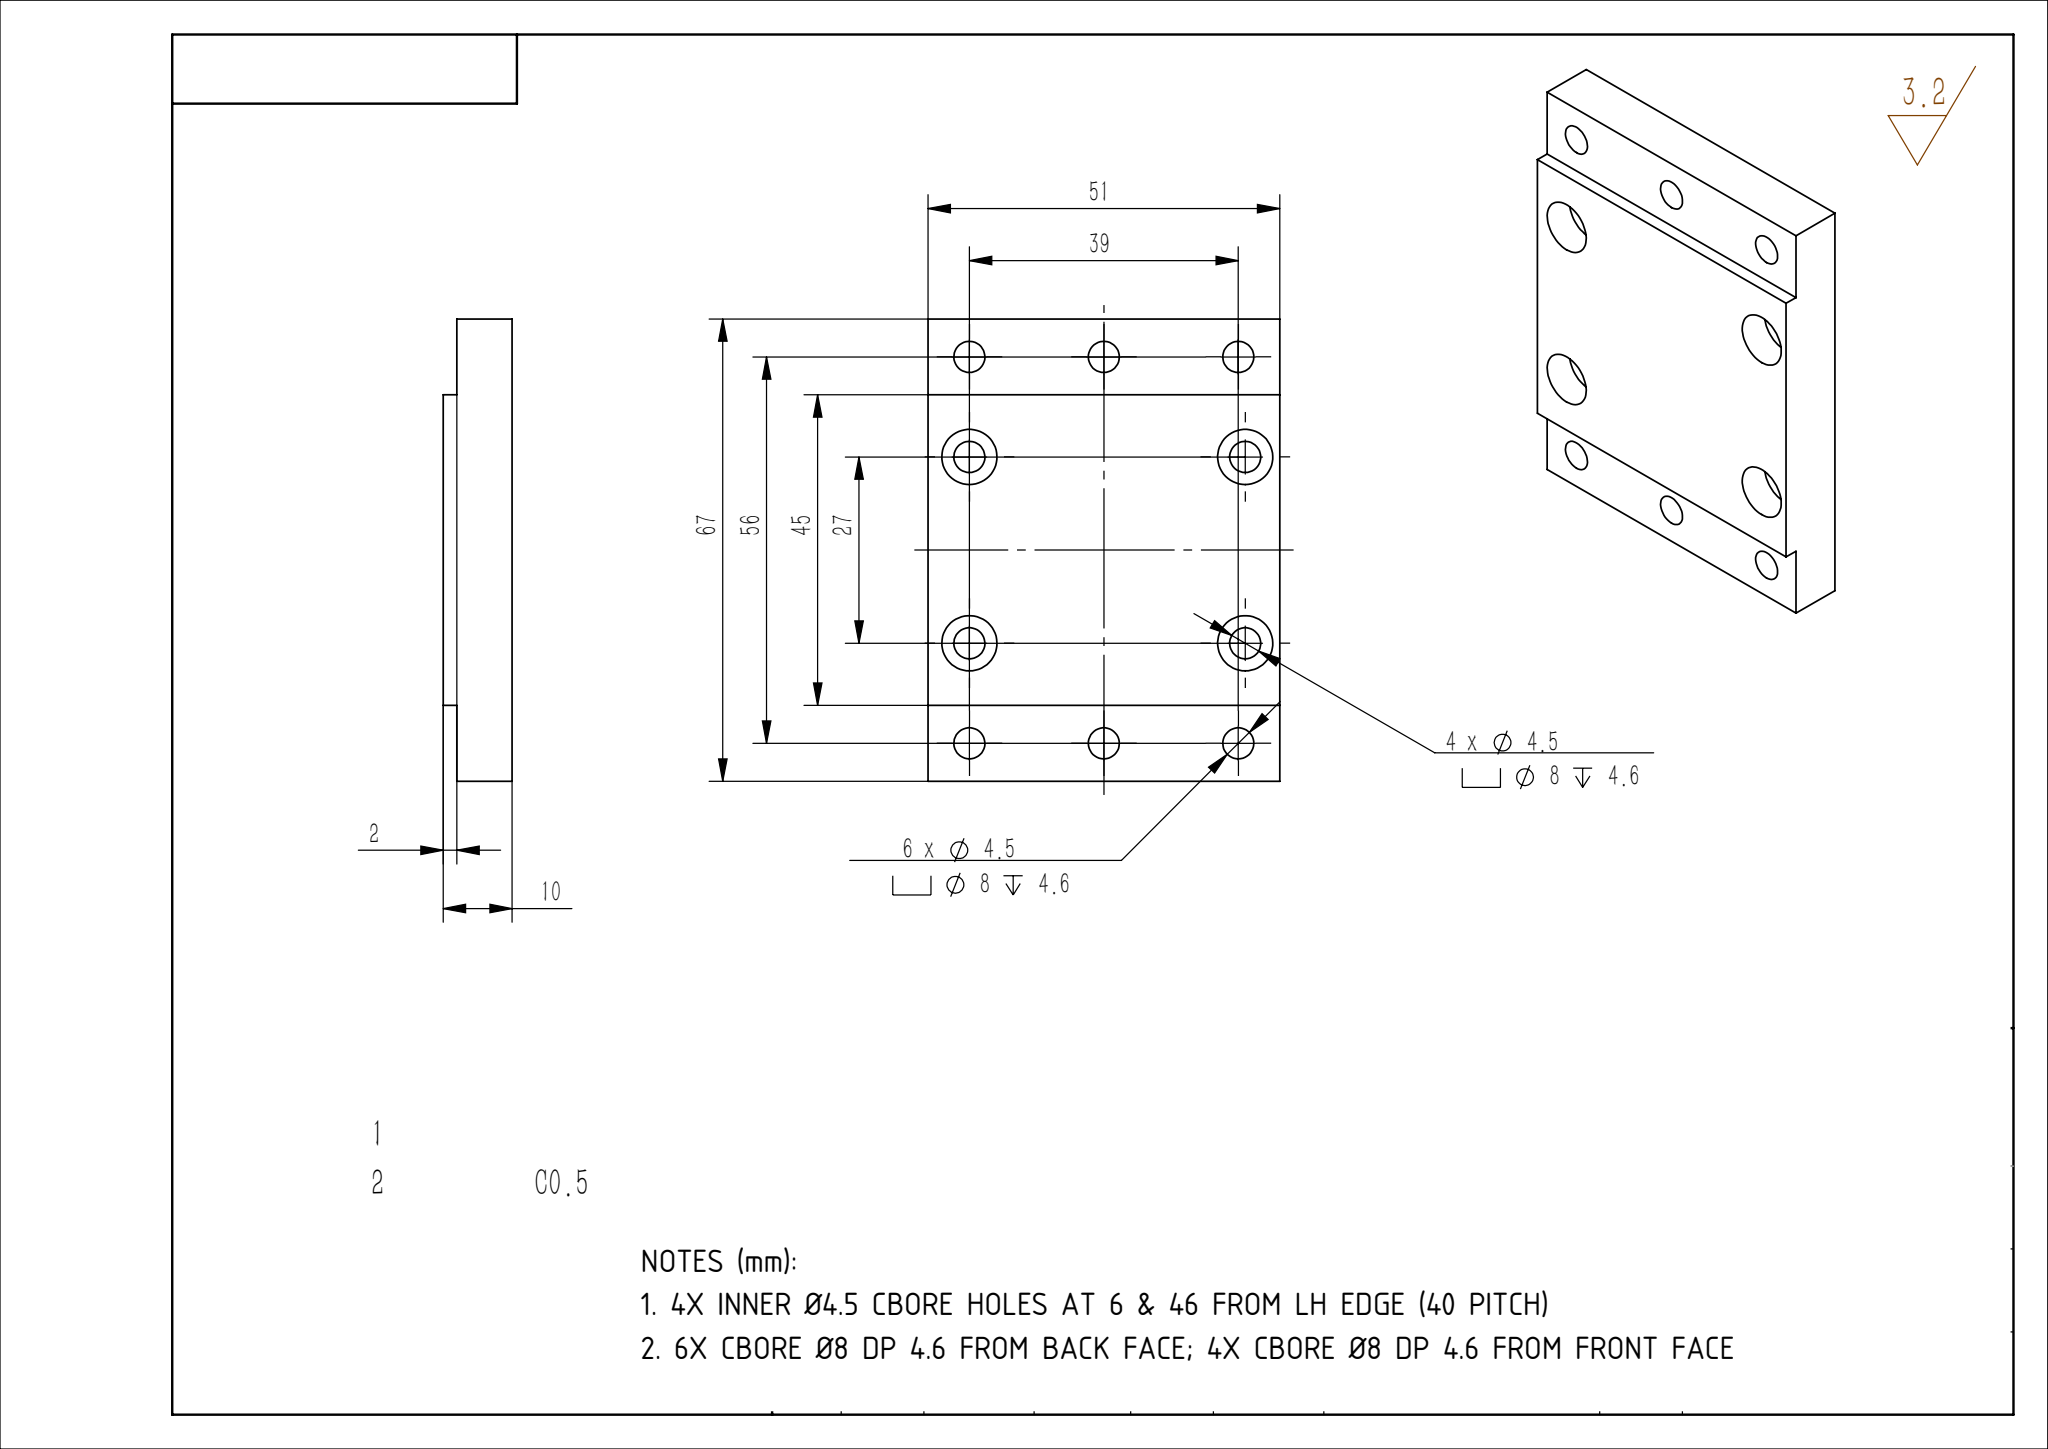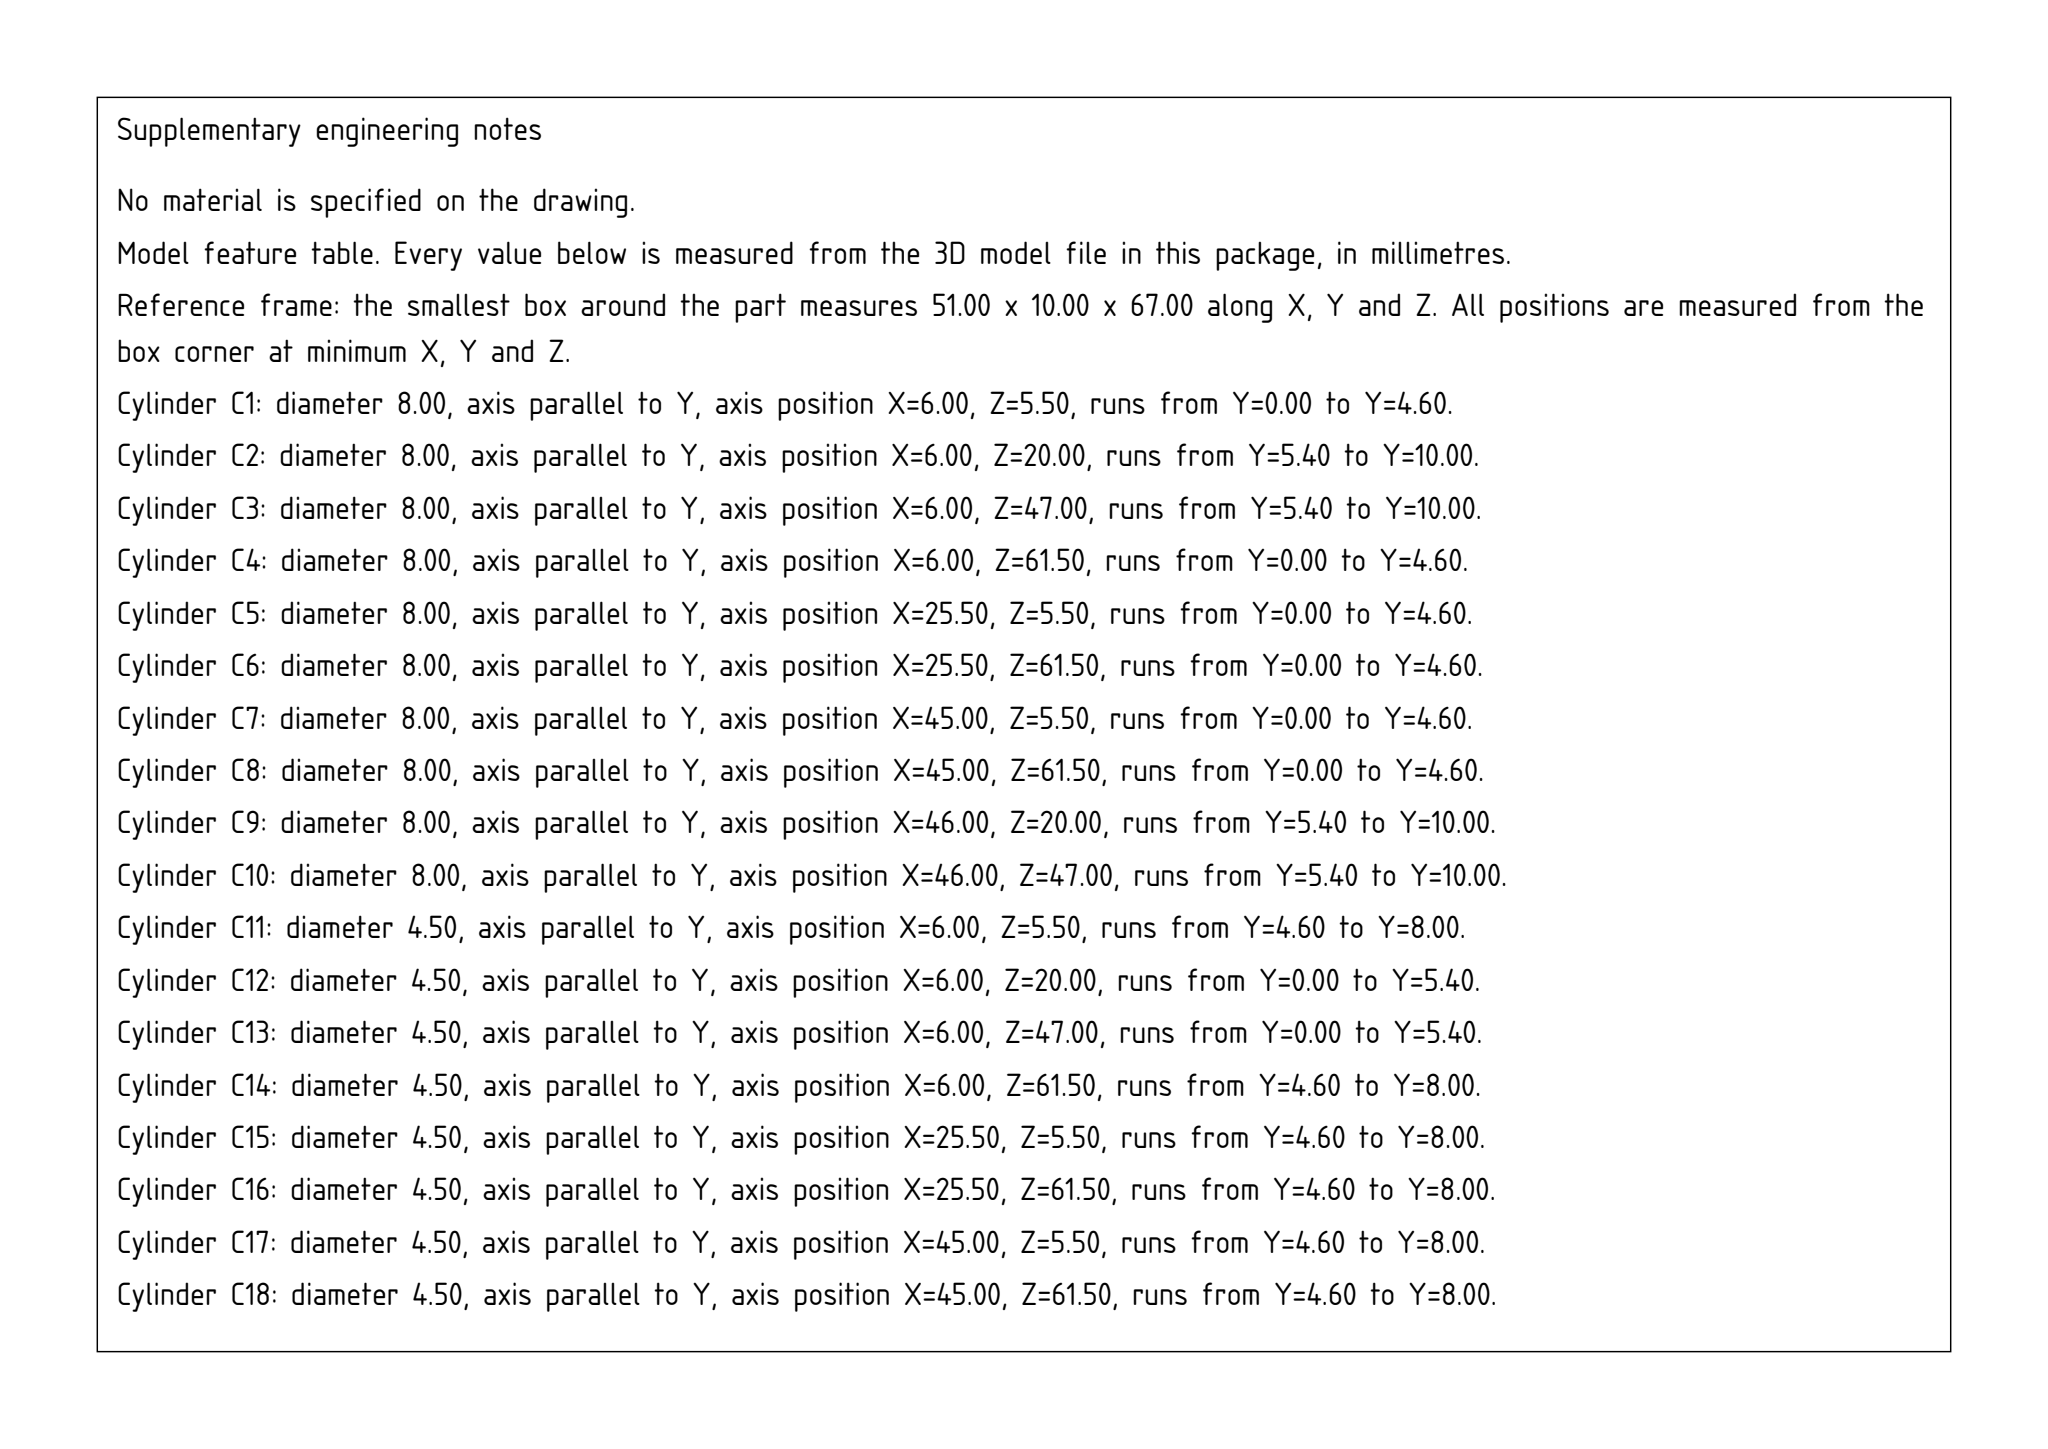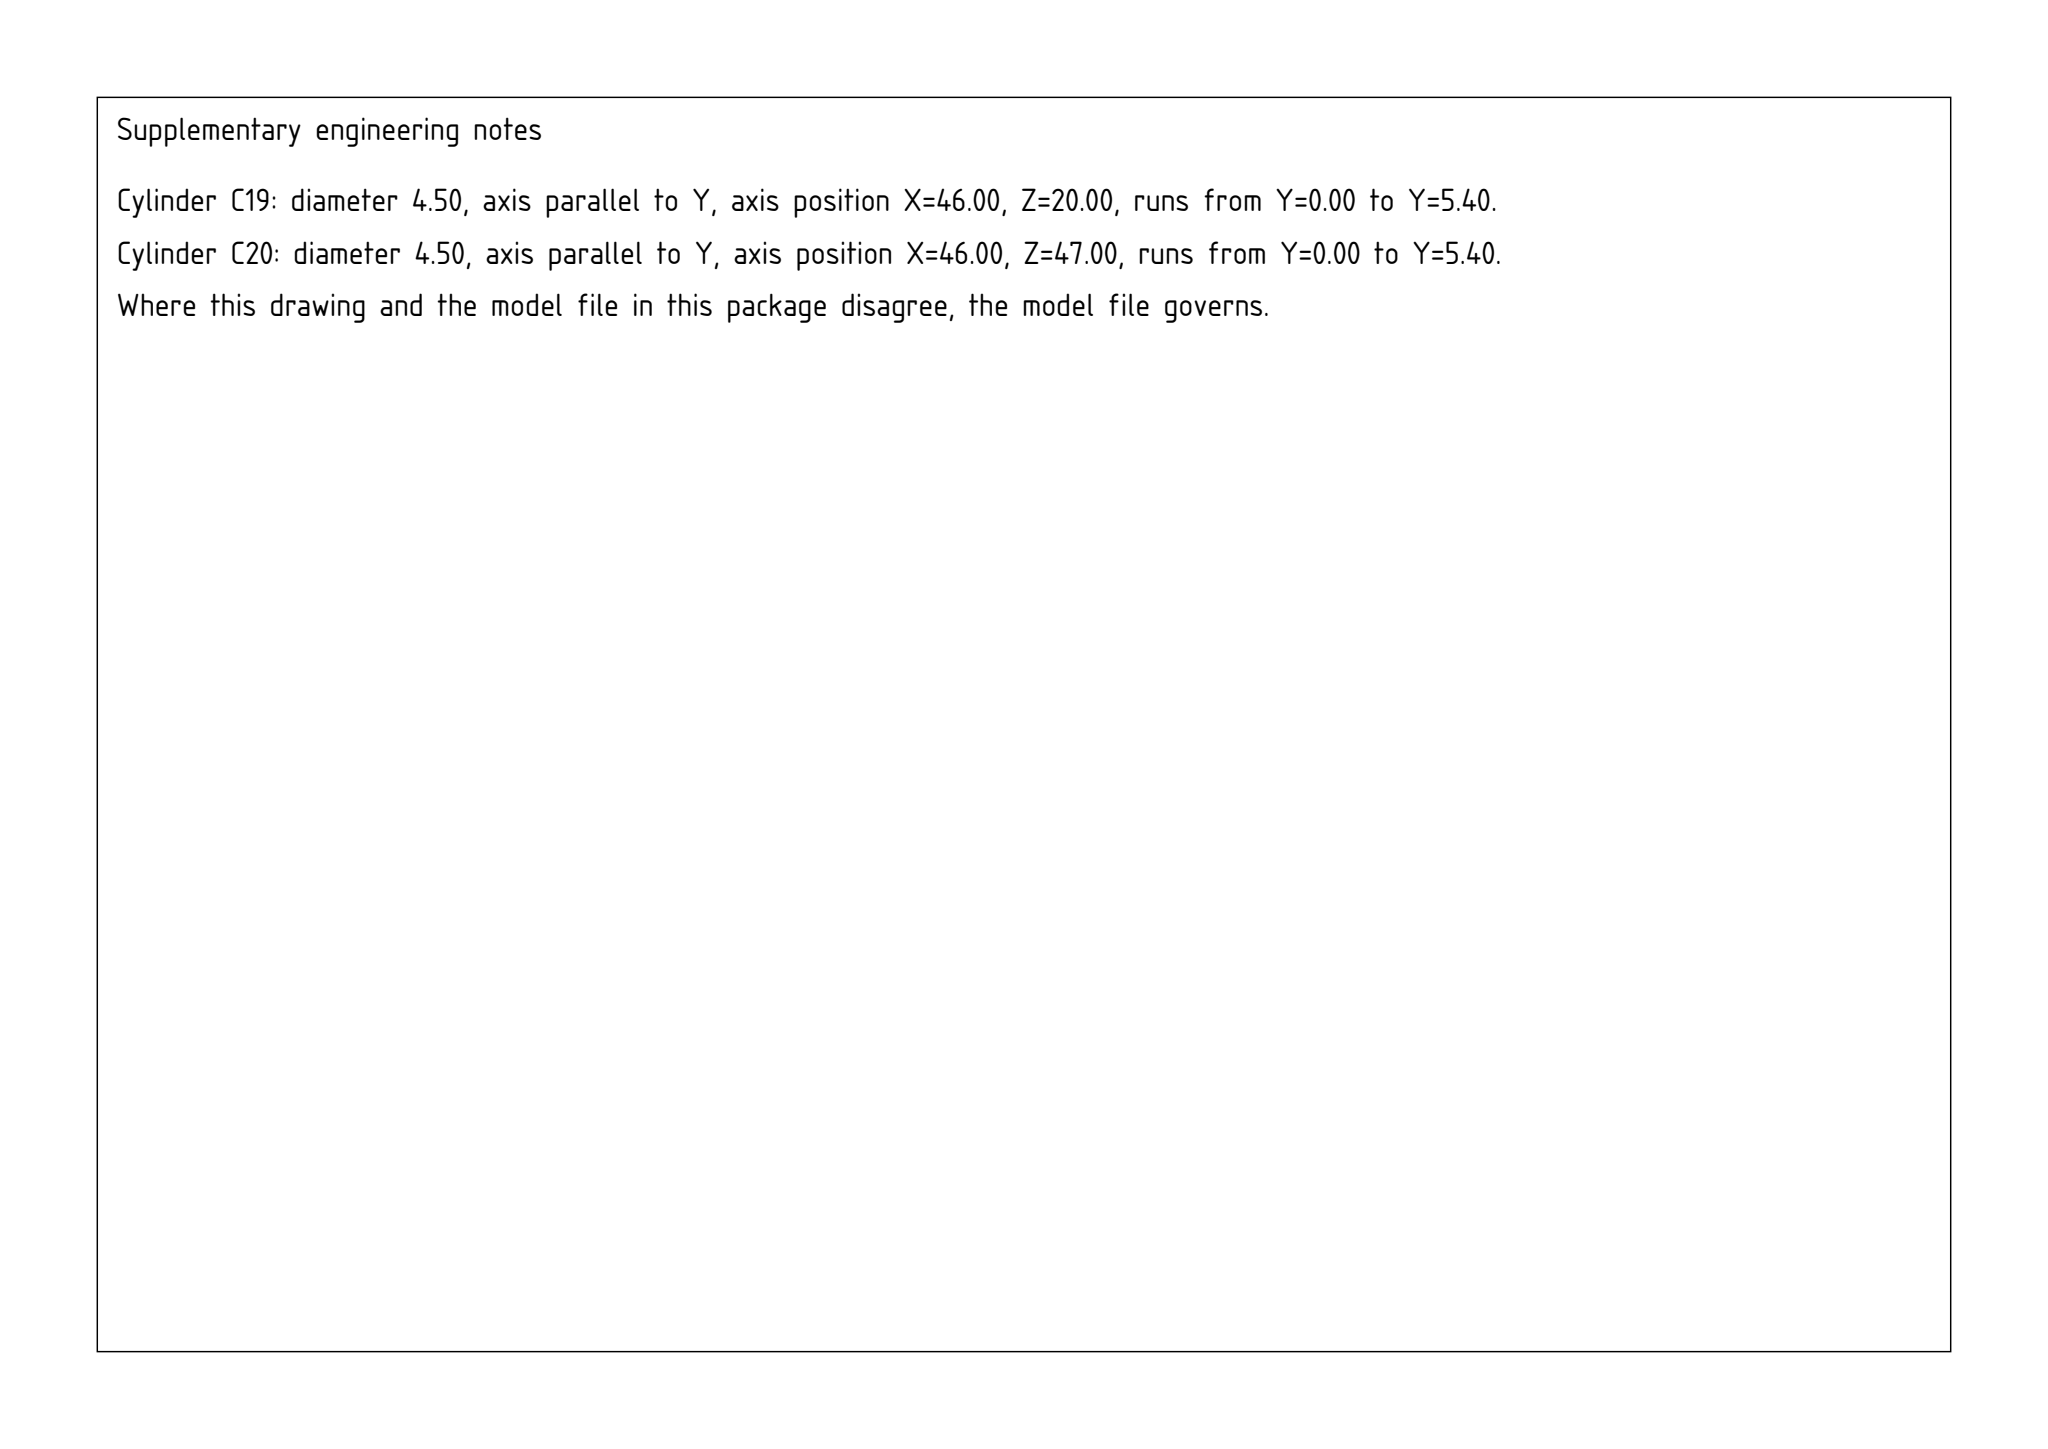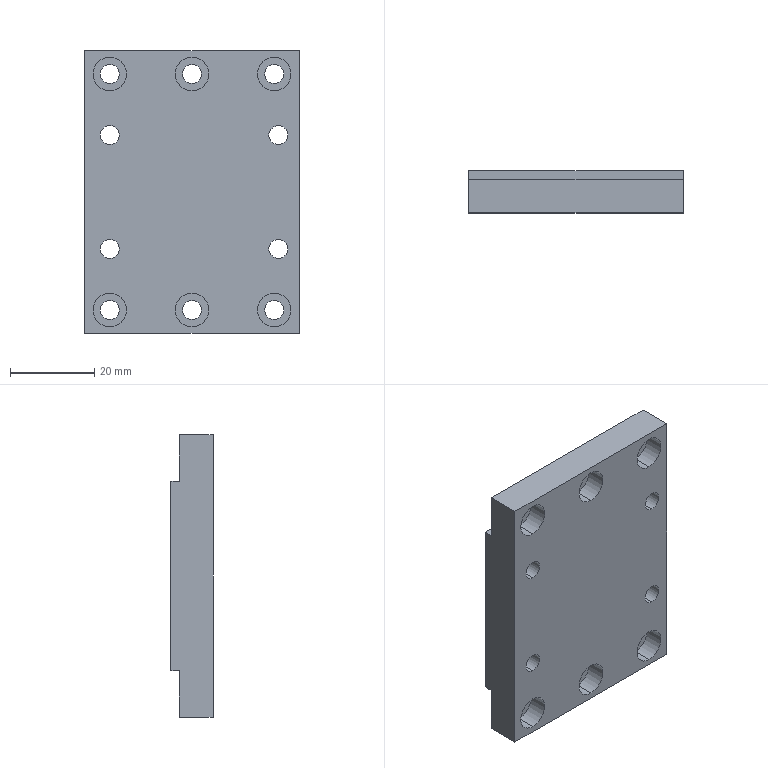Part | SolidWorks | mm | 1 solid | 60 faces | box 51 x 10 x 67 mm | volume 28946 mm3 | cylinder 40 | plane 20 | commonest cylinder face diameters 8 x20 4.5 x20
Drawing notes:
4X INNER Ø4.5 CBORE HOLES AT 6 & 46 FROM LH EDGE (40 PITCH) | from the solid: Ø4.5/Ø8 holes at x=6.0 and x=46.0 (z=20,47); bbox X=51, so 46 = 5 from RH edge, 40 pitch
6X CBORE Ø8 DP 4.6 FROM BACK FACE; 4X CBORE Ø8 DP 4.6 FROM FRONT FACE | from the solid: 6 cbore bottoms at y=4.6 (from y=0 face), 4 cbore bottoms at y=5.4 (from y=10 face)
build123d program:
from build123d import *

# Parameters (mm, degrees)
SKETCH1_W                                         = 51
SKETCH1_H                                         = 67
BOSS_EXTRUDE1_DEPTH                               = 10
SKETCH2_W                                         = 51
SKETCH2_H                                         = 11
CUT_EXTRUDE1_DEPTH                                = 2
HOLE_SIZE_ACCORDING_TO_TYPE_2_OF_HEXA_D           = 4.5
HOLE_SIZE_ACCORDING_TO_TYPE_2_OF_HEXA_CBORE_D     = 8
HOLE_SIZE_ACCORDING_TO_TYPE_2_OF_HEXA_CBORE_DEPTH = 4.6
HOLE_SIZE_ACCORDING_TO_TYPE_2_OF_2_D              = 4.5
HOLE_SIZE_ACCORDING_TO_TYPE_2_OF_2_CBORE_D        = 8
HOLE_SIZE_ACCORDING_TO_TYPE_2_OF_2_CBORE_DEPTH    = 4.6


with BuildPart() as part:
    # Sketch1 → Boss-Extrude1 (new body)
    with BuildSketch(Plane(origin=(0, 0, 0), x_dir=(1, 0, 0), z_dir=(0, 1, 0))):
        Rectangle(SKETCH1_W, SKETCH1_H)
    extrude(amount=BOSS_EXTRUDE1_DEPTH)

    # Sketch2 → Cut-Extrude1 (cut)
    with BuildSketch(Plane(origin=(0, 10, 0), x_dir=(1, 0, 0), z_dir=(0, 1, 0))):
        with Locations((0, 28)):
            Rectangle(SKETCH2_W, SKETCH2_H)
        with Locations((0, -28)):
            Rectangle(SKETCH2_W, SKETCH2_H)
    extrude(amount=-CUT_EXTRUDE1_DEPTH, mode=Mode.SUBTRACT)

    # Hole Size _ according to_ type 2 of Hexa (through all)
    with Locations(Plane(origin=(0, 10, 0), x_dir=(1, 0, 0), z_dir=(0, 1, 0))):
        with Locations((-19.5, 13.5), (20.5, 13.5)):
            hole_size_according_to_type_2_of_hexa = CounterBoreHole(HOLE_SIZE_ACCORDING_TO_TYPE_2_OF_HEXA_D / 2, HOLE_SIZE_ACCORDING_TO_TYPE_2_OF_HEXA_CBORE_D / 2, HOLE_SIZE_ACCORDING_TO_TYPE_2_OF_HEXA_CBORE_DEPTH)

    # Hole Size _ according to_ type 2 of  2 (through all)
    with Locations(Plane(origin=(0, 0, 0), x_dir=(-1, 0, 0), z_dir=(0, -1, 0))):
        with Locations((-19.5, 28), (0, 28), (19.5, 28)):
            hole_size_according_to_type_2_of_2 = CounterBoreHole(HOLE_SIZE_ACCORDING_TO_TYPE_2_OF_2_D / 2, HOLE_SIZE_ACCORDING_TO_TYPE_2_OF_2_CBORE_D / 2, HOLE_SIZE_ACCORDING_TO_TYPE_2_OF_2_CBORE_DEPTH)

    # Mirror1: Hole Size _ according to_ type 2 of Hexa, Hole Size _ according to_ type 2 of  2 across plane
    add(hole_size_according_to_type_2_of_hexa.mirror(Plane.XY), mode=Mode.SUBTRACT)
    add(hole_size_according_to_type_2_of_2.mirror(Plane.XY), mode=Mode.SUBTRACT)


solid = part.part